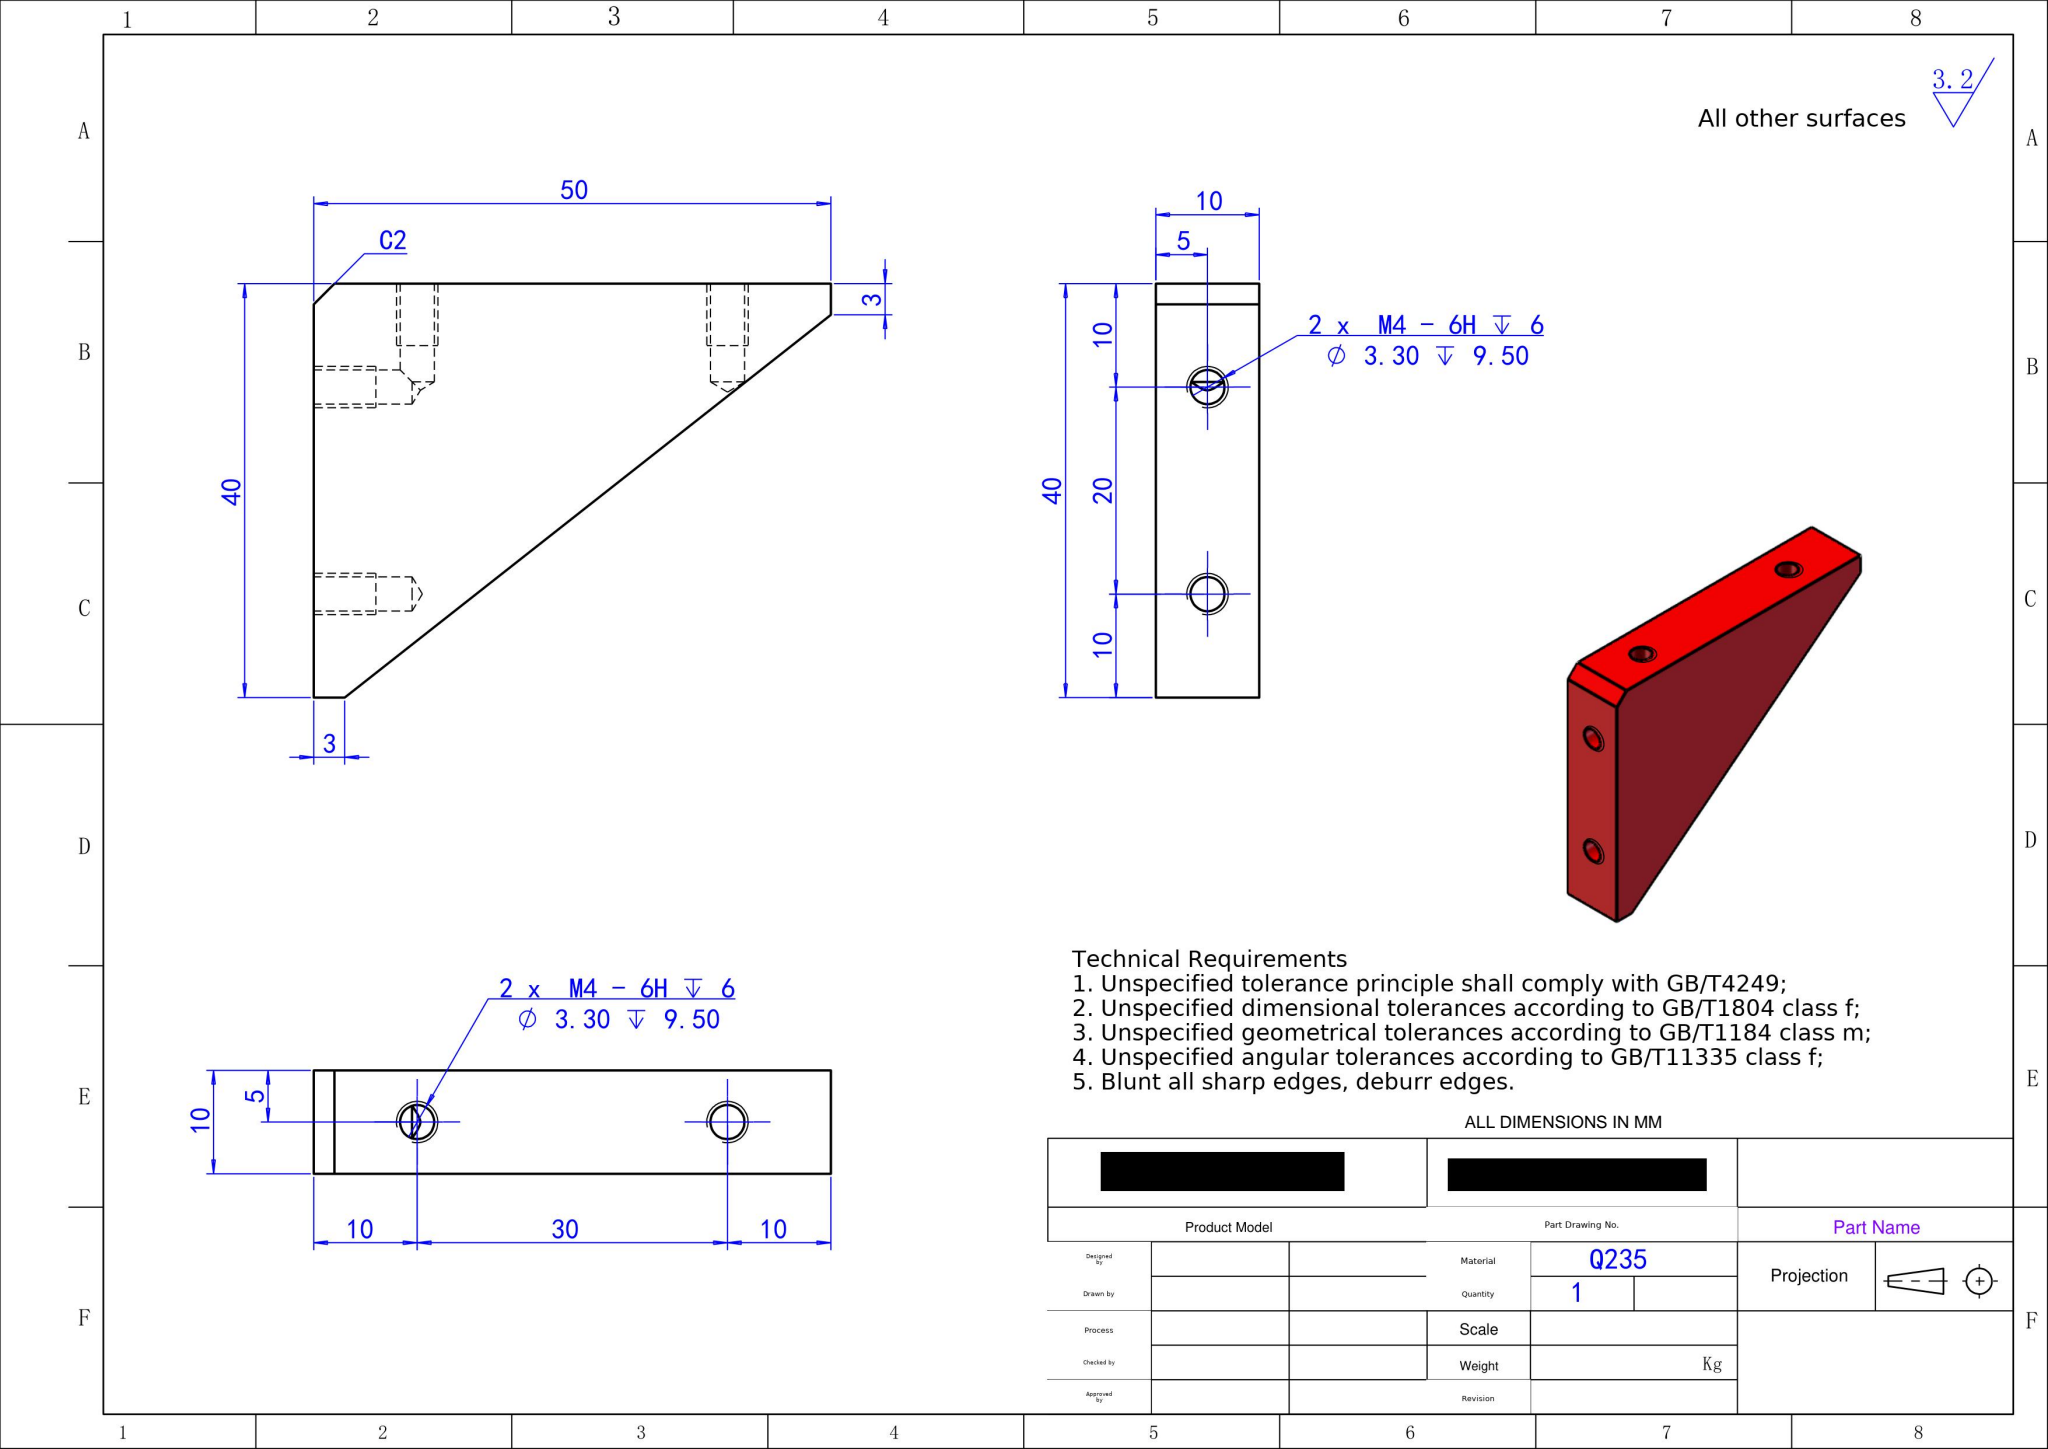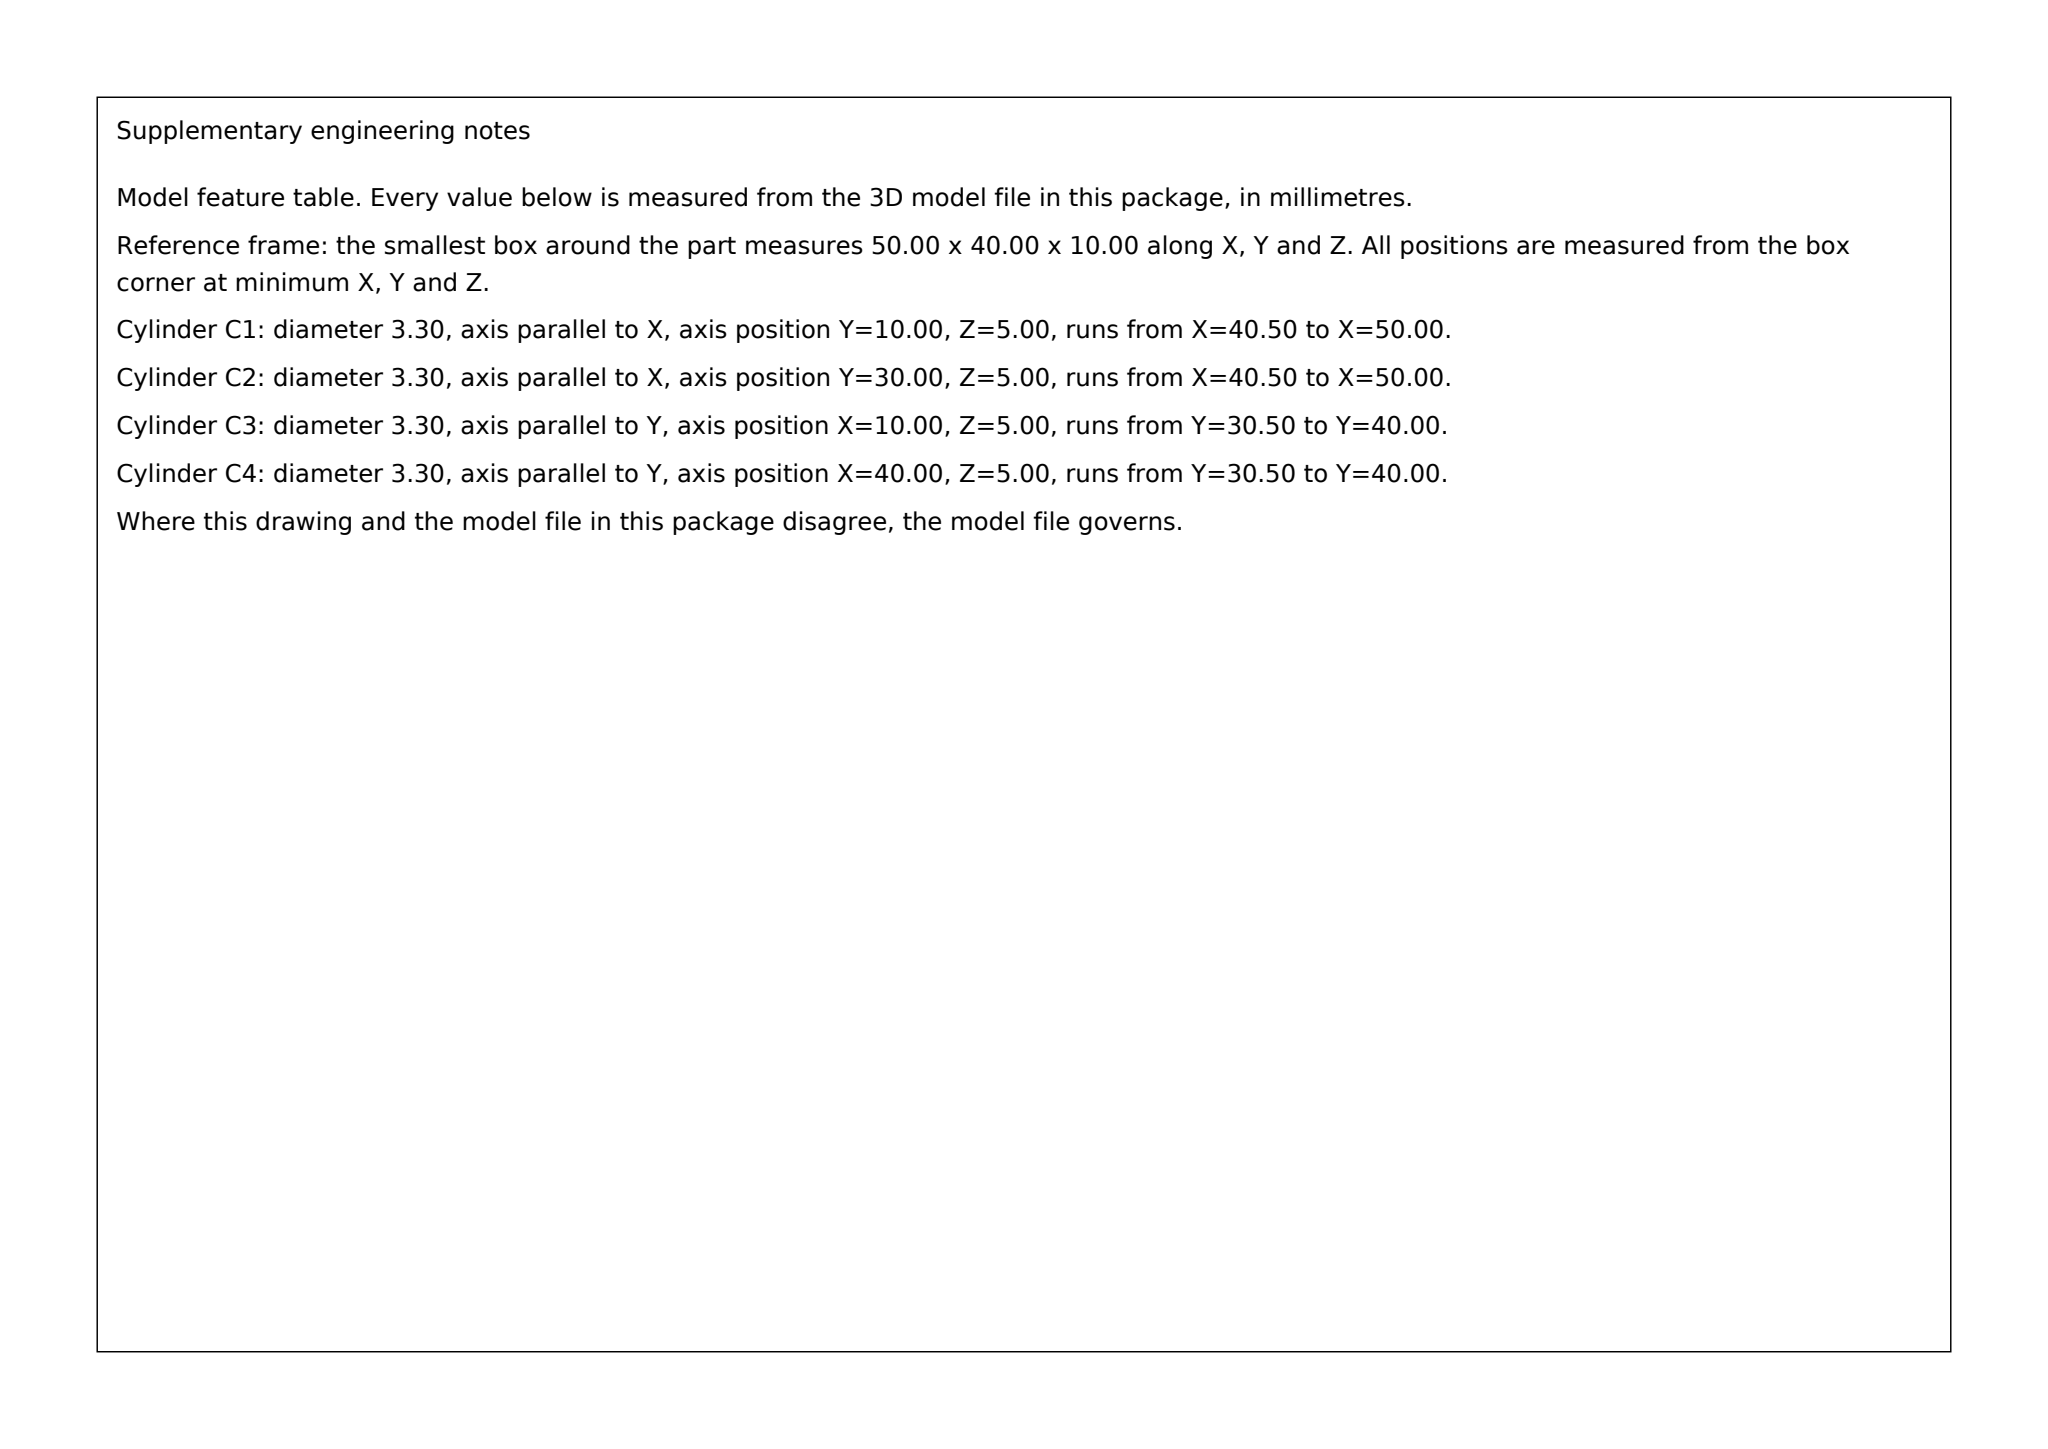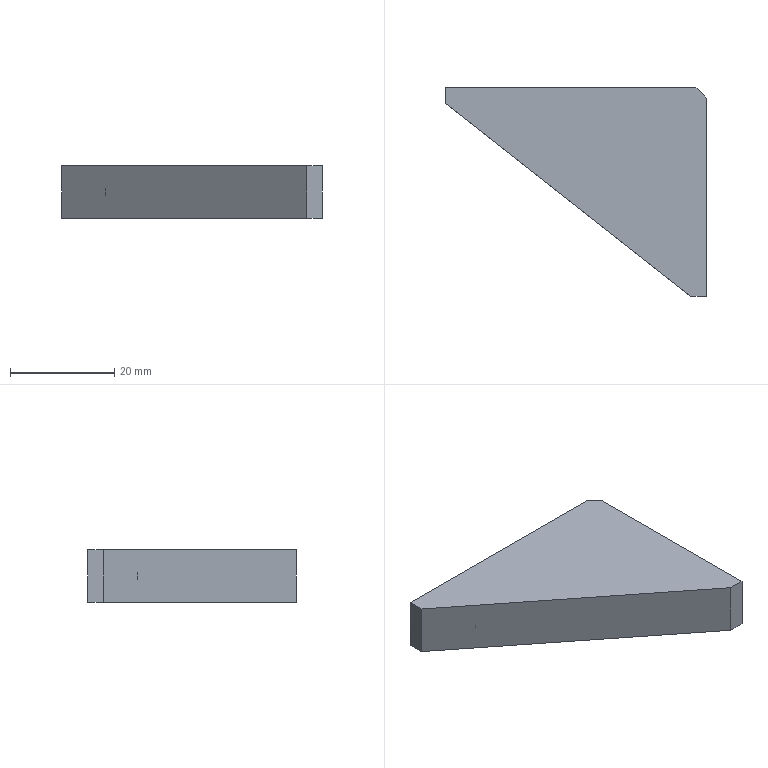Part | SolidWorks | mm | 1 solid | 26 faces | box 50 x 40 x 10 mm | volume 10953 mm3 | cone 10 | cylinder 8 | plane 8 | commonest cylinder face diameters 3.3 x8
build123d program:
from build123d import *

# Parameters (mm, degrees)
BOSS_EXTRUDE1_DEPTH   = 5
M4_TAPPED_HOLE1_D     = 3.3
M4_TAPPED_HOLE1_DEPTH = 9.5
M4_TAPPED_HOLE1_TIP   = 0.9914
M4_TAPPED_HOLE2_D     = 3.3
M4_TAPPED_HOLE2_DEPTH = 9.5
M4_TAPPED_HOLE2_TIP   = 0.9914
CHAMFER1_SIZE         = 2


with BuildPart() as part:
    # Sketch1 → Boss-Extrude1 (new, symmetric)
    with BuildSketch(Plane.XY):
        Polygon((-50, 0), (-50, -3), (-3, -40), (0, -40), (0, 0), align=None)
    extrude(amount=BOSS_EXTRUDE1_DEPTH, both=True)

    # M4 Tapped Hole1
    with Locations(Plane(origin=(0, 0, 0), x_dir=(1, 0, 0), z_dir=(0, 1, 0))):
        with Locations((-40, 0), (-10, 0)):
            Hole(M4_TAPPED_HOLE1_D / 2, depth=M4_TAPPED_HOLE1_DEPTH)
            with Locations((0, 0, -(M4_TAPPED_HOLE1_DEPTH + M4_TAPPED_HOLE1_TIP / 2))):  # 118° drill point
                Cone(0, M4_TAPPED_HOLE1_D / 2, M4_TAPPED_HOLE1_TIP, mode=Mode.SUBTRACT)

    # M4 Tapped Hole2
    with Locations(Plane(origin=(0, 0, 0), x_dir=(0, 0, -1), z_dir=(1, 0, 0))):
        with Locations((0, -10), (0, -30)):
            Hole(M4_TAPPED_HOLE2_D / 2, depth=M4_TAPPED_HOLE2_DEPTH)
            with Locations((0, 0, -(M4_TAPPED_HOLE2_DEPTH + M4_TAPPED_HOLE2_TIP / 2))):  # 118° drill point
                Cone(0, M4_TAPPED_HOLE2_D / 2, M4_TAPPED_HOLE2_TIP, mode=Mode.SUBTRACT)

    # Chamfer1
    chamfer1_edges = [part.edges().sort_by_distance(p)[0] for p in [
        (0, 0, 0),
    ]]
    chamfer(chamfer1_edges, length=CHAMFER1_SIZE)


solid = part.part
STEP:
#1=CARTESIAN_POINT('',(-10.,-10.,0.8179));
#2=VERTEX_POINT('',#1);
#3=CARTESIAN_POINT('',(-10.,-10.,-0.8179));
#4=VERTEX_POINT('',#3);
#5=CARTESIAN_POINT('',(-10.,-10.,0.8179));
#6=CARTESIAN_POINT('',(-10.072,-10.072,0.6979));
#7=CARTESIAN_POINT('',(-10.142,-10.142,0.5744));
#8=CARTESIAN_POINT('',(-10.23,-10.23,0.3745));
#9=CARTESIAN_POINT('',(-10.256,-10.256,0.3058));
#10=CARTESIAN_POINT('',(-10.294,-10.294,0.1596));
#11=CARTESIAN_POINT('',(-10.307,-10.307,0.08021));
#12=CARTESIAN_POINT('',(-10.307,-10.307,-0.07708));
#13=CARTESIAN_POINT('',(-10.295,-10.295,-0.1564));
#14=CARTESIAN_POINT('',(-10.256,-10.256,-0.3047));
#15=CARTESIAN_POINT('',(-10.229,-10.229,-0.3753));
#16=CARTESIAN_POINT('',(-10.141,-10.141,-0.5754));
#17=CARTESIAN_POINT('',(-10.072,-10.072,-0.698));
#18=CARTESIAN_POINT('',(-10.,-10.,-0.8179));
#19=B_SPLINE_CURVE_WITH_KNOTS('',3,(#5,#6,#7,#8,#9,#10,#11,#12,#13,#14,#15,#16,#17,#18),.UNSPECIFIED.,.F.,.F.,(4,2,2,2,2,2,4),(0.001035,0.001506,0.001742,0.001978,0.002213,0.002449,0.002921),.UNSPECIFIED.);
#20=EDGE_CURVE('',#2,#4,#19,.T.);
#21=ORIENTED_EDGE('',*,*,#20,.F.);
#22=CARTESIAN_POINT('',(-9.5,-10.,1.65));
#23=VERTEX_POINT('',#22);
#24=CARTESIAN_POINT('',(-9.5,-10.,1.65));
#25=DIRECTION('',(0.515,0.,0.8572));
#26=VECTOR('',#25,1000.);
#27=LINE('',#24,#26);
#28=EDGE_CURVE('',#2,#23,#27,.T.);
#29=ORIENTED_EDGE('',*,*,#28,.T.);
#30=CARTESIAN_POINT('',(-9.5,-10.,-1.65));
#31=VERTEX_POINT('',#30);
#32=CARTESIAN_POINT('',(-9.5,-10.,0.));
#33=DIRECTION('',(1.,0.,0.));
#34=DIRECTION('',(0.,0.,-1.));
#35=AXIS2_PLACEMENT_3D('',#32,#33,#34);
#36=CIRCLE('',#35,1.65);
#37=EDGE_CURVE('',#23,#31,#36,.T.);
#38=ORIENTED_EDGE('',*,*,#37,.T.);
#39=CARTESIAN_POINT('',(-9.5,-10.,-1.65));
#40=DIRECTION('',(0.515,0.,-0.8572));
#41=VECTOR('',#40,1000.);
#42=LINE('',#39,#41);
#43=EDGE_CURVE('',#4,#31,#42,.T.);
#44=ORIENTED_EDGE('',*,*,#43,.F.);
#45=EDGE_LOOP('',(#21,#29,#38,#44));
#46=FACE_OUTER_BOUND('',#45,.T.);
#47=CARTESIAN_POINT('',(-9.5,-10.,0.));
#48=DIRECTION('',(1.,0.,0.));
#49=DIRECTION('',(0.,0.,-1.));
#50=AXIS2_PLACEMENT_3D('',#47,#48,#49);
#51=CONICAL_SURFACE('',#50,1.65,1.03);
#52=ADVANCED_FACE('',(#46),#51,.F.);
#53=CARTESIAN_POINT('',(-9.5,-9.5,-1.572));
#54=VERTEX_POINT('',#53);
#55=CARTESIAN_POINT('',(-10.,-10.,-0.8179));
#56=CARTESIAN_POINT('',(-9.842,-9.842,-1.081));
#57=CARTESIAN_POINT('',(-9.672,-9.672,-1.327));
#58=CARTESIAN_POINT('',(-9.5,-9.5,-1.572));
#59=B_SPLINE_CURVE_WITH_KNOTS('',3,(#55,#56,#57,#58),.UNSPECIFIED.,.F.,.F.,(4,4),(0.002921,0.003954),.UNSPECIFIED.);
#60=EDGE_CURVE('',#4,#54,#59,.T.);
#61=ORIENTED_EDGE('',*,*,#60,.F.);
#62=ORIENTED_EDGE('',*,*,#43,.T.);
#63=CARTESIAN_POINT('',(-9.5,-10.,0.));
#64=DIRECTION('',(1.,0.,0.));
#65=DIRECTION('',(0.,0.,-1.));
#66=AXIS2_PLACEMENT_3D('',#63,#64,#65);
#67=CIRCLE('',#66,1.65);
#68=EDGE_CURVE('',#31,#54,#67,.T.);
#69=ORIENTED_EDGE('',*,*,#68,.T.);
#70=EDGE_LOOP('',(#61,#62,#69));
#71=FACE_OUTER_BOUND('',#70,.T.);
#72=CARTESIAN_POINT('',(-9.5,-10.,0.));
#73=DIRECTION('',(1.,0.,0.));
#74=DIRECTION('',(0.,0.,-1.));
#75=AXIS2_PLACEMENT_3D('',#72,#73,#74);
#76=CONICAL_SURFACE('',#75,1.65,1.03);
#77=ADVANCED_FACE('',(#71),#76,.F.);
#78=ORIENTED_EDGE('',*,*,#37,.F.);
#79=CARTESIAN_POINT('',(0.,-10.,1.65));
#80=VERTEX_POINT('',#79);
#81=CARTESIAN_POINT('',(0.,-10.,1.65));
#82=DIRECTION('',(1.,0.,0.));
#83=VECTOR('',#82,1000.);
#84=LINE('',#81,#83);
#85=EDGE_CURVE('',#23,#80,#84,.T.);
#86=ORIENTED_EDGE('',*,*,#85,.T.);
#87=CARTESIAN_POINT('',(0.,-10.,-1.65));
#88=VERTEX_POINT('',#87);
#89=CARTESIAN_POINT('',(0.,-10.,0.));
#90=DIRECTION('',(1.,0.,0.));
#91=DIRECTION('',(0.,0.,-1.));
#92=AXIS2_PLACEMENT_3D('',#89,#90,#91);
#93=CIRCLE('',#92,1.65);
#94=EDGE_CURVE('',#80,#88,#93,.T.);
#95=ORIENTED_EDGE('',*,*,#94,.T.);
#96=CARTESIAN_POINT('',(0.,-10.,-1.65));
#97=DIRECTION('',(1.,0.,0.));
#98=VECTOR('',#97,1000.);
#99=LINE('',#96,#98);
#100=EDGE_CURVE('',#31,#88,#99,.T.);
#101=ORIENTED_EDGE('',*,*,#100,.F.);
#102=EDGE_LOOP('',(#78,#86,#95,#101));
#103=FACE_OUTER_BOUND('',#102,.T.);
#104=CARTESIAN_POINT('',(0.,-10.,0.));
#105=DIRECTION('',(1.,0.,0.));
#106=DIRECTION('',(0.,0.,-1.));
#107=AXIS2_PLACEMENT_3D('',#104,#105,#106);
#108=CYLINDRICAL_SURFACE('',#107,1.65);
#109=ADVANCED_FACE('',(#103),#108,.F.);
#110=CARTESIAN_POINT('',(-9.5,-30.,1.65));
#111=VERTEX_POINT('',#110);
#112=CARTESIAN_POINT('',(-9.5,-30.,-1.65));
#113=VERTEX_POINT('',#112);
#114=CARTESIAN_POINT('',(-9.5,-30.,0.));
#115=DIRECTION('',(1.,0.,0.));
#116=DIRECTION('',(0.,0.,-1.));
#117=AXIS2_PLACEMENT_3D('',#114,#115,#116);
#118=CIRCLE('',#117,1.65);
#119=EDGE_CURVE('',#111,#113,#118,.T.);
#120=ORIENTED_EDGE('',*,*,#119,.F.);
#121=CARTESIAN_POINT('',(0.,-30.,1.65));
#122=VERTEX_POINT('',#121);
#123=CARTESIAN_POINT('',(0.,-30.,1.65));
#124=DIRECTION('',(1.,0.,0.));
#125=VECTOR('',#124,1000.);
#126=LINE('',#123,#125);
#127=EDGE_CURVE('',#111,#122,#126,.T.);
#128=ORIENTED_EDGE('',*,*,#127,.T.);
#129=CARTESIAN_POINT('',(0.,-30.,-1.65));
#130=VERTEX_POINT('',#129);
#131=CARTESIAN_POINT('',(0.,-30.,0.));
#132=DIRECTION('',(1.,0.,0.));
#133=DIRECTION('',(0.,0.,-1.));
#134=AXIS2_PLACEMENT_3D('',#131,#132,#133);
#135=CIRCLE('',#134,1.65);
#136=EDGE_CURVE('',#122,#130,#135,.T.);
#137=ORIENTED_EDGE('',*,*,#136,.T.);
#138=CARTESIAN_POINT('',(0.,-30.,-1.65));
#139=DIRECTION('',(1.,0.,0.));
#140=VECTOR('',#139,1000.);
#141=LINE('',#138,#140);
#142=EDGE_CURVE('',#113,#130,#141,.T.);
#143=ORIENTED_EDGE('',*,*,#142,.F.);
#144=EDGE_LOOP('',(#120,#128,#137,#143));
#145=FACE_OUTER_BOUND('',#144,.T.);
#146=CARTESIAN_POINT('',(0.,-30.,0.));
#147=DIRECTION('',(1.,0.,0.));
#148=DIRECTION('',(0.,0.,-1.));
#149=AXIS2_PLACEMENT_3D('',#146,#147,#148);
#150=CYLINDRICAL_SURFACE('',#149,1.65);
#151=ADVANCED_FACE('',(#145),#150,.F.);
#152=CARTESIAN_POINT('',(-10.491,-30.,0.));
#153=VERTEX_POINT('',#152);
#154=CARTESIAN_POINT('',(-9.5,-30.,-1.65));
#155=DIRECTION('',(0.515,0.,-0.8572));
#156=VECTOR('',#155,1000.);
#157=LINE('',#154,#156);
#158=EDGE_CURVE('',#153,#113,#157,.T.);
#159=ORIENTED_EDGE('',*,*,#158,.F.);
#160=CARTESIAN_POINT('',(-9.5,-30.,1.65));
#161=DIRECTION('',(0.515,0.,0.8572));
#162=VECTOR('',#161,1000.);
#163=LINE('',#160,#162);
#164=EDGE_CURVE('',#153,#111,#163,.T.);
#165=ORIENTED_EDGE('',*,*,#164,.T.);
#166=ORIENTED_EDGE('',*,*,#119,.T.);
#167=EDGE_LOOP('',(#159,#165,#166));
#168=FACE_OUTER_BOUND('',#167,.T.);
#169=CARTESIAN_POINT('',(-9.5,-30.,0.));
#170=DIRECTION('',(1.,0.,0.));
#171=DIRECTION('',(0.,0.,-1.));
#172=AXIS2_PLACEMENT_3D('',#169,#170,#171);
#173=CONICAL_SURFACE('',#172,1.65,1.03);
#174=ADVANCED_FACE('',(#168),#173,.F.);
#175=CARTESIAN_POINT('',(-40.,-9.5,-1.65));
#176=VERTEX_POINT('',#175);
#177=CARTESIAN_POINT('',(-40.,-9.5,1.65));
#178=VERTEX_POINT('',#177);
#179=CARTESIAN_POINT('',(-40.,-9.5,0.));
#180=DIRECTION('',(0.,1.,0.));
#181=DIRECTION('',(0.,0.,1.));
#182=AXIS2_PLACEMENT_3D('',#179,#180,#181);
#183=CIRCLE('',#182,1.65);
#184=EDGE_CURVE('',#176,#178,#183,.T.);
#185=ORIENTED_EDGE('',*,*,#184,.F.);
#186=CARTESIAN_POINT('',(-40.,-0.,-1.65));
#187=VERTEX_POINT('',#186);
#188=CARTESIAN_POINT('',(-40.,-0.,-1.65));
#189=DIRECTION('',(0.,1.,0.));
#190=VECTOR('',#189,1000.);
#191=LINE('',#188,#190);
#192=EDGE_CURVE('',#176,#187,#191,.T.);
#193=ORIENTED_EDGE('',*,*,#192,.T.);
#194=CARTESIAN_POINT('',(-40.,-0.,1.65));
#195=VERTEX_POINT('',#194);
#196=CARTESIAN_POINT('',(-40.,-0.,0.));
#197=DIRECTION('',(0.,1.,0.));
#198=DIRECTION('',(0.,0.,1.));
#199=AXIS2_PLACEMENT_3D('',#196,#197,#198);
#200=CIRCLE('',#199,1.65);
#201=EDGE_CURVE('',#187,#195,#200,.T.);
#202=ORIENTED_EDGE('',*,*,#201,.T.);
#203=CARTESIAN_POINT('',(-40.,-0.,1.65));
#204=DIRECTION('',(0.,1.,0.));
#205=VECTOR('',#204,1000.);
#206=LINE('',#203,#205);
#207=EDGE_CURVE('',#178,#195,#206,.T.);
#208=ORIENTED_EDGE('',*,*,#207,.F.);
#209=EDGE_LOOP('',(#185,#193,#202,#208));
#210=FACE_OUTER_BOUND('',#209,.T.);
#211=CARTESIAN_POINT('',(-40.,-0.,0.));
#212=DIRECTION('',(0.,1.,0.));
#213=DIRECTION('',(0.,0.,1.));
#214=AXIS2_PLACEMENT_3D('',#211,#212,#213);
#215=CYLINDRICAL_SURFACE('',#214,1.65);
#216=ADVANCED_FACE('',(#210),#215,.F.);
#217=CARTESIAN_POINT('',(-40.,-10.491,0.));
#218=VERTEX_POINT('',#217);
#219=CARTESIAN_POINT('',(-40.,-9.5,1.65));
#220=DIRECTION('',(0.,0.515,0.8572));
#221=VECTOR('',#220,1000.);
#222=LINE('',#219,#221);
#223=EDGE_CURVE('',#218,#178,#222,.T.);
#224=ORIENTED_EDGE('',*,*,#223,.F.);
#225=CARTESIAN_POINT('',(-40.,-9.5,-1.65));
#226=DIRECTION('',(0.,0.515,-0.8572));
#227=VECTOR('',#226,1000.);
#228=LINE('',#225,#227);
#229=EDGE_CURVE('',#218,#176,#228,.T.);
#230=ORIENTED_EDGE('',*,*,#229,.T.);
#231=ORIENTED_EDGE('',*,*,#184,.T.);
#232=EDGE_LOOP('',(#224,#230,#231));
#233=FACE_OUTER_BOUND('',#232,.T.);
#234=CARTESIAN_POINT('',(-40.,-9.5,0.));
#235=DIRECTION('',(0.,1.,0.));
#236=DIRECTION('',(0.,0.,1.));
#237=AXIS2_PLACEMENT_3D('',#234,#235,#236);
#238=CONICAL_SURFACE('',#237,1.65,1.03);
#239=ADVANCED_FACE('',(#233),#238,.F.);
#240=CARTESIAN_POINT('',(-10.,-9.5,-1.65));
#241=VERTEX_POINT('',#240);
#242=CARTESIAN_POINT('',(-10.,-9.5,1.65));
#243=VERTEX_POINT('',#242);
#244=CARTESIAN_POINT('',(-10.,-9.5,0.));
#245=DIRECTION('',(0.,1.,0.));
#246=DIRECTION('',(0.,0.,1.));
#247=AXIS2_PLACEMENT_3D('',#244,#245,#246);
#248=CIRCLE('',#247,1.65);
#249=EDGE_CURVE('',#241,#243,#248,.T.);
#250=ORIENTED_EDGE('',*,*,#249,.F.);
#251=CARTESIAN_POINT('',(-10.,0.,-1.65));
#252=VERTEX_POINT('',#251);
#253=CARTESIAN_POINT('',(-10.,0.,-1.65));
#254=DIRECTION('',(0.,1.,0.));
#255=VECTOR('',#254,1000.);
#256=LINE('',#253,#255);
#257=EDGE_CURVE('',#241,#252,#256,.T.);
#258=ORIENTED_EDGE('',*,*,#257,.T.);
#259=CARTESIAN_POINT('',(-10.,0.,1.65));
#260=VERTEX_POINT('',#259);
#261=CARTESIAN_POINT('',(-10.,0.,0.));
#262=DIRECTION('',(0.,1.,0.));
#263=DIRECTION('',(0.,0.,1.));
#264=AXIS2_PLACEMENT_3D('',#261,#262,#263);
#265=CIRCLE('',#264,1.65);
#266=EDGE_CURVE('',#252,#260,#265,.T.);
#267=ORIENTED_EDGE('',*,*,#266,.T.);
#268=CARTESIAN_POINT('',(-10.,0.,1.65));
#269=DIRECTION('',(0.,1.,0.));
#270=VECTOR('',#269,1000.);
#271=LINE('',#268,#270);
#272=EDGE_CURVE('',#243,#260,#271,.T.);
#273=ORIENTED_EDGE('',*,*,#272,.F.);
#274=EDGE_LOOP('',(#250,#258,#267,#273));
#275=FACE_OUTER_BOUND('',#274,.T.);
#276=CARTESIAN_POINT('',(-10.,0.,0.));
#277=DIRECTION('',(0.,1.,0.));
#278=DIRECTION('',(0.,0.,1.));
#279=AXIS2_PLACEMENT_3D('',#276,#277,#278);
#280=CYLINDRICAL_SURFACE('',#279,1.65);
#281=ADVANCED_FACE('',(#275),#280,.F.);
#282=ORIENTED_EDGE('',*,*,#20,.T.);
#283=CARTESIAN_POINT('',(-10.,-9.5,-1.65));
#284=DIRECTION('',(0.,0.515,-0.8572));
#285=VECTOR('',#284,1000.);
#286=LINE('',#283,#285);
#287=EDGE_CURVE('',#4,#241,#286,.T.);
#288=ORIENTED_EDGE('',*,*,#287,.T.);
#289=ORIENTED_EDGE('',*,*,#249,.T.);
#290=CARTESIAN_POINT('',(-10.,-9.5,1.65));
#291=DIRECTION('',(0.,0.515,0.8572));
#292=VECTOR('',#291,1000.);
#293=LINE('',#290,#292);
#294=EDGE_CURVE('',#2,#243,#293,.T.);
#295=ORIENTED_EDGE('',*,*,#294,.F.);
#296=EDGE_LOOP('',(#282,#288,#289,#295));
#297=FACE_OUTER_BOUND('',#296,.T.);
#298=CARTESIAN_POINT('',(-10.,-9.5,0.));
#299=DIRECTION('',(0.,1.,0.));
#300=DIRECTION('',(0.,0.,1.));
#301=AXIS2_PLACEMENT_3D('',#298,#299,#300);
#302=CONICAL_SURFACE('',#301,1.65,1.03);
#303=ADVANCED_FACE('',(#297),#302,.F.);
#304=CARTESIAN_POINT('',(-9.5,-9.5,1.572));
#305=VERTEX_POINT('',#304);
#306=CARTESIAN_POINT('',(-9.5,-9.5,1.572));
#307=CARTESIAN_POINT('',(-9.672,-9.672,1.327));
#308=CARTESIAN_POINT('',(-9.842,-9.842,1.081));
#309=CARTESIAN_POINT('',(-10.,-10.,0.8179));
#310=B_SPLINE_CURVE_WITH_KNOTS('',3,(#306,#307,#308,#309),.UNSPECIFIED.,.F.,.F.,(4,4),(0.0000004,0.001035),.UNSPECIFIED.);
#311=EDGE_CURVE('',#305,#2,#310,.T.);
#312=ORIENTED_EDGE('',*,*,#311,.T.);
#313=ORIENTED_EDGE('',*,*,#294,.T.);
#314=CARTESIAN_POINT('',(-10.,-9.5,0.));
#315=DIRECTION('',(0.,1.,0.));
#316=DIRECTION('',(0.,0.,1.));
#317=AXIS2_PLACEMENT_3D('',#314,#315,#316);
#318=CIRCLE('',#317,1.65);
#319=EDGE_CURVE('',#243,#305,#318,.T.);
#320=ORIENTED_EDGE('',*,*,#319,.T.);
#321=EDGE_LOOP('',(#312,#313,#320));
#322=FACE_OUTER_BOUND('',#321,.T.);
#323=CARTESIAN_POINT('',(-10.,-9.5,0.));
#324=DIRECTION('',(0.,1.,0.));
#325=DIRECTION('',(0.,0.,1.));
#326=AXIS2_PLACEMENT_3D('',#323,#324,#325);
#327=CONICAL_SURFACE('',#326,1.65,1.03);
#328=ADVANCED_FACE('',(#322),#327,.F.);
#329=CARTESIAN_POINT('',(-40.,-0.,0.));
#330=DIRECTION('',(0.,1.,0.));
#331=DIRECTION('',(0.,0.,1.));
#332=AXIS2_PLACEMENT_3D('',#329,#330,#331);
#333=CIRCLE('',#332,1.65);
#334=EDGE_CURVE('',#195,#187,#333,.T.);
#335=ORIENTED_EDGE('',*,*,#334,.F.);
#336=ORIENTED_EDGE('',*,*,#201,.F.);
#337=EDGE_LOOP('',(#335,#336));
#338=FACE_BOUND('',#337,.T.);
#339=CARTESIAN_POINT('',(-10.,0.,0.));
#340=DIRECTION('',(0.,1.,0.));
#341=DIRECTION('',(0.,0.,1.));
#342=AXIS2_PLACEMENT_3D('',#339,#340,#341);
#343=CIRCLE('',#342,1.65);
#344=EDGE_CURVE('',#260,#252,#343,.T.);
#345=ORIENTED_EDGE('',*,*,#344,.F.);
#346=ORIENTED_EDGE('',*,*,#266,.F.);
#347=EDGE_LOOP('',(#345,#346));
#348=FACE_BOUND('',#347,.T.);
#349=CARTESIAN_POINT('',(-2.,0.,5.));
#350=VERTEX_POINT('',#349);
#351=CARTESIAN_POINT('',(-50.,-0.,5.));
#352=VERTEX_POINT('',#351);
#353=CARTESIAN_POINT('',(0.,0.,5.));
#354=DIRECTION('',(-1.,-0.,0.));
#355=VECTOR('',#354,1000.);
#356=LINE('',#353,#355);
#357=EDGE_CURVE('',#350,#352,#356,.T.);
#358=ORIENTED_EDGE('',*,*,#357,.F.);
#359=CARTESIAN_POINT('',(-2.,0.,-5.));
#360=VERTEX_POINT('',#359);
#361=CARTESIAN_POINT('',(-2.,0.,-5.));
#362=DIRECTION('',(0.,0.,-1.));
#363=VECTOR('',#362,1000.);
#364=LINE('',#361,#363);
#365=EDGE_CURVE('',#350,#360,#364,.T.);
#366=ORIENTED_EDGE('',*,*,#365,.T.);
#367=CARTESIAN_POINT('',(-50.,-0.,-5.));
#368=VERTEX_POINT('',#367);
#369=CARTESIAN_POINT('',(0.,0.,-5.));
#370=DIRECTION('',(-1.,-0.,0.));
#371=VECTOR('',#370,1000.);
#372=LINE('',#369,#371);
#373=EDGE_CURVE('',#360,#368,#372,.T.);
#374=ORIENTED_EDGE('',*,*,#373,.T.);
#375=CARTESIAN_POINT('',(-50.,-0.,5.));
#376=DIRECTION('',(0.,0.,-1.));
#377=VECTOR('',#376,1000.);
#378=LINE('',#375,#377);
#379=EDGE_CURVE('',#352,#368,#378,.T.);
#380=ORIENTED_EDGE('',*,*,#379,.F.);
#381=EDGE_LOOP('',(#358,#366,#374,#380));
#382=FACE_OUTER_BOUND('',#381,.T.);
#383=CARTESIAN_POINT('',(0.,0.,5.));
#384=DIRECTION('',(0.,-1.,0.));
#385=DIRECTION('',(1.,0.,0.));
#386=AXIS2_PLACEMENT_3D('',#383,#384,#385);
#387=PLANE('',#386);
#388=ADVANCED_FACE('',(#338,#348,#382),#387,.F.);
#389=CARTESIAN_POINT('',(-50.,-3.,-5.));
#390=VERTEX_POINT('',#389);
#391=CARTESIAN_POINT('',(-50.,-0.,-5.));
#392=DIRECTION('',(0.,-1.,0.));
#393=VECTOR('',#392,1000.);
#394=LINE('',#391,#393);
#395=EDGE_CURVE('',#368,#390,#394,.T.);
#396=ORIENTED_EDGE('',*,*,#395,.T.);
#397=CARTESIAN_POINT('',(-50.,-3.,5.));
#398=VERTEX_POINT('',#397);
#399=CARTESIAN_POINT('',(-50.,-3.,5.));
#400=DIRECTION('',(0.,0.,-1.));
#401=VECTOR('',#400,1000.);
#402=LINE('',#399,#401);
#403=EDGE_CURVE('',#398,#390,#402,.T.);
#404=ORIENTED_EDGE('',*,*,#403,.F.);
#405=CARTESIAN_POINT('',(-50.,-0.,5.));
#406=DIRECTION('',(0.,-1.,0.));
#407=VECTOR('',#406,1000.);
#408=LINE('',#405,#407);
#409=EDGE_CURVE('',#352,#398,#408,.T.);
#410=ORIENTED_EDGE('',*,*,#409,.F.);
#411=ORIENTED_EDGE('',*,*,#379,.T.);
#412=EDGE_LOOP('',(#396,#404,#410,#411));
#413=FACE_OUTER_BOUND('',#412,.T.);
#414=CARTESIAN_POINT('',(-50.,-0.,5.));
#415=DIRECTION('',(1.,0.,0.));
#416=DIRECTION('',(-0.,1.,0.));
#417=AXIS2_PLACEMENT_3D('',#414,#415,#416);
#418=PLANE('',#417);
#419=ADVANCED_FACE('',(#413),#418,.F.);
#420=CARTESIAN_POINT('',(-3.,-40.,-5.));
#421=VERTEX_POINT('',#420);
#422=CARTESIAN_POINT('',(-20.589,-26.153,-5.));
#423=DIRECTION('',(0.7857,-0.6186,0.));
#424=VECTOR('',#423,1000.);
#425=LINE('',#422,#424);
#426=EDGE_CURVE('',#390,#421,#425,.T.);
#427=ORIENTED_EDGE('',*,*,#426,.T.);
#428=CARTESIAN_POINT('',(-3.,-40.,5.));
#429=VERTEX_POINT('',#428);
#430=CARTESIAN_POINT('',(-3.,-40.,5.));
#431=DIRECTION('',(0.,0.,-1.));
#432=VECTOR('',#431,1000.);
#433=LINE('',#430,#432);
#434=EDGE_CURVE('',#429,#421,#433,.T.);
#435=ORIENTED_EDGE('',*,*,#434,.F.);
#436=CARTESIAN_POINT('',(-20.589,-26.153,5.));
#437=DIRECTION('',(0.7857,-0.6186,0.));
#438=VECTOR('',#437,1000.);
#439=LINE('',#436,#438);
#440=EDGE_CURVE('',#398,#429,#439,.T.);
#441=ORIENTED_EDGE('',*,*,#440,.F.);
#442=ORIENTED_EDGE('',*,*,#403,.T.);
#443=EDGE_LOOP('',(#427,#435,#441,#442));
#444=FACE_OUTER_BOUND('',#443,.T.);
#445=CARTESIAN_POINT('',(-20.589,-26.153,5.));
#446=DIRECTION('',(0.6186,0.7857,0.));
#447=DIRECTION('',(-0.7857,0.6186,0.));
#448=AXIS2_PLACEMENT_3D('',#445,#446,#447);
#449=PLANE('',#448);
#450=ADVANCED_FACE('',(#444),#449,.F.);
#451=CARTESIAN_POINT('',(0.,-40.,-5.));
#452=VERTEX_POINT('',#451);
#453=CARTESIAN_POINT('',(0.,-40.,-5.));
#454=DIRECTION('',(-1.,-0.,0.));
#455=VECTOR('',#454,1000.);
#456=LINE('',#453,#455);
#457=EDGE_CURVE('',#452,#421,#456,.T.);
#458=ORIENTED_EDGE('',*,*,#457,.F.);
#459=CARTESIAN_POINT('',(0.,-40.,5.));
#460=VERTEX_POINT('',#459);
#461=CARTESIAN_POINT('',(0.,-40.,5.));
#462=DIRECTION('',(0.,0.,-1.));
#463=VECTOR('',#462,1000.);
#464=LINE('',#461,#463);
#465=EDGE_CURVE('',#460,#452,#464,.T.);
#466=ORIENTED_EDGE('',*,*,#465,.F.);
#467=CARTESIAN_POINT('',(0.,-40.,5.));
#468=DIRECTION('',(-1.,-0.,0.));
#469=VECTOR('',#468,1000.);
#470=LINE('',#467,#469);
#471=EDGE_CURVE('',#460,#429,#470,.T.);
#472=ORIENTED_EDGE('',*,*,#471,.T.);
#473=ORIENTED_EDGE('',*,*,#434,.T.);
#474=EDGE_LOOP('',(#458,#466,#472,#473));
#475=FACE_OUTER_BOUND('',#474,.T.);
#476=CARTESIAN_POINT('',(0.,-40.,5.));
#477=DIRECTION('',(0.,-1.,0.));
#478=DIRECTION('',(1.,0.,0.));
#479=AXIS2_PLACEMENT_3D('',#476,#477,#478);
#480=PLANE('',#479);
#481=ADVANCED_FACE('',(#475),#480,.T.);
#482=CARTESIAN_POINT('',(0.,-10.,0.));
#483=DIRECTION('',(1.,0.,0.));
#484=DIRECTION('',(0.,0.,-1.));
#485=AXIS2_PLACEMENT_3D('',#482,#483,#484);
#486=CIRCLE('',#485,1.65);
#487=EDGE_CURVE('',#88,#80,#486,.T.);
#488=ORIENTED_EDGE('',*,*,#487,.F.);
#489=ORIENTED_EDGE('',*,*,#94,.F.);
#490=EDGE_LOOP('',(#488,#489));
#491=FACE_BOUND('',#490,.T.);
#492=CARTESIAN_POINT('',(0.,-30.,0.));
#493=DIRECTION('',(1.,0.,0.));
#494=DIRECTION('',(0.,0.,-1.));
#495=AXIS2_PLACEMENT_3D('',#492,#493,#494);
#496=CIRCLE('',#495,1.65);
#497=EDGE_CURVE('',#130,#122,#496,.T.);
#498=ORIENTED_EDGE('',*,*,#497,.F.);
#499=ORIENTED_EDGE('',*,*,#136,.F.);
#500=EDGE_LOOP('',(#498,#499));
#501=FACE_BOUND('',#500,.T.);
#502=CARTESIAN_POINT('',(0.,-2.,-5.));
#503=VERTEX_POINT('',#502);
#504=CARTESIAN_POINT('',(0.,0.,-5.));
#505=DIRECTION('',(0.,-1.,0.));
#506=VECTOR('',#505,1000.);
#507=LINE('',#504,#506);
#508=EDGE_CURVE('',#503,#452,#507,.T.);
#509=ORIENTED_EDGE('',*,*,#508,.F.);
#510=CARTESIAN_POINT('',(0.,-2.,5.));
#511=VERTEX_POINT('',#510);
#512=CARTESIAN_POINT('',(0.,-2.,5.));
#513=DIRECTION('',(0.,0.,1.));
#514=VECTOR('',#513,1000.);
#515=LINE('',#512,#514);
#516=EDGE_CURVE('',#503,#511,#515,.T.);
#517=ORIENTED_EDGE('',*,*,#516,.T.);
#518=CARTESIAN_POINT('',(0.,0.,5.));
#519=DIRECTION('',(0.,-1.,0.));
#520=VECTOR('',#519,1000.);
#521=LINE('',#518,#520);
#522=EDGE_CURVE('',#511,#460,#521,.T.);
#523=ORIENTED_EDGE('',*,*,#522,.T.);
#524=ORIENTED_EDGE('',*,*,#465,.T.);
#525=EDGE_LOOP('',(#509,#517,#523,#524));
#526=FACE_OUTER_BOUND('',#525,.T.);
#527=CARTESIAN_POINT('',(0.,0.,5.));
#528=DIRECTION('',(1.,0.,0.));
#529=DIRECTION('',(-0.,1.,0.));
#530=AXIS2_PLACEMENT_3D('',#527,#528,#529);
#531=PLANE('',#530);
#532=ADVANCED_FACE('',(#491,#501,#526),#531,.T.);
#533=ORIENTED_EDGE('',*,*,#522,.F.);
#534=CARTESIAN_POINT('',(-1.,-1.,5.));
#535=DIRECTION('',(-0.7071,0.7071,0.));
#536=VECTOR('',#535,1000.);
#537=LINE('',#534,#536);
#538=EDGE_CURVE('',#511,#350,#537,.T.);
#539=ORIENTED_EDGE('',*,*,#538,.T.);
#540=ORIENTED_EDGE('',*,*,#357,.T.);
#541=ORIENTED_EDGE('',*,*,#409,.T.);
#542=ORIENTED_EDGE('',*,*,#440,.T.);
#543=ORIENTED_EDGE('',*,*,#471,.F.);
#544=EDGE_LOOP('',(#533,#539,#540,#541,#542,#543));
#545=FACE_OUTER_BOUND('',#544,.T.);
#546=CARTESIAN_POINT('',(0.,0.,5.));
#547=DIRECTION('',(0.,0.,1.));
#548=DIRECTION('',(1.,0.,0.));
#549=AXIS2_PLACEMENT_3D('',#546,#547,#548);
#550=PLANE('',#549);
#551=ADVANCED_FACE('',(#545),#550,.T.);
#552=ORIENTED_EDGE('',*,*,#373,.F.);
#553=CARTESIAN_POINT('',(-2.,0.,-5.));
#554=DIRECTION('',(0.7071,-0.7071,0.));
#555=VECTOR('',#554,1000.);
#556=LINE('',#553,#555);
#557=EDGE_CURVE('',#360,#503,#556,.T.);
#558=ORIENTED_EDGE('',*,*,#557,.T.);
#559=ORIENTED_EDGE('',*,*,#508,.T.);
#560=ORIENTED_EDGE('',*,*,#457,.T.);
#561=ORIENTED_EDGE('',*,*,#426,.F.);
#562=ORIENTED_EDGE('',*,*,#395,.F.);
#563=EDGE_LOOP('',(#552,#558,#559,#560,#561,#562));
#564=FACE_OUTER_BOUND('',#563,.T.);
#565=CARTESIAN_POINT('',(0.,0.,-5.));
#566=DIRECTION('',(0.,0.,1.));
#567=DIRECTION('',(1.,0.,0.));
#568=AXIS2_PLACEMENT_3D('',#565,#566,#567);
#569=PLANE('',#568);
#570=ADVANCED_FACE('',(#564),#569,.F.);
#571=ORIENTED_EDGE('',*,*,#287,.F.);
#572=ORIENTED_EDGE('',*,*,#60,.T.);
#573=CARTESIAN_POINT('',(-10.,-9.5,0.));
#574=DIRECTION('',(0.,1.,0.));
#575=DIRECTION('',(0.,0.,1.));
#576=AXIS2_PLACEMENT_3D('',#573,#574,#575);
#577=CIRCLE('',#576,1.65);
#578=EDGE_CURVE('',#54,#241,#577,.T.);
#579=ORIENTED_EDGE('',*,*,#578,.T.);
#580=EDGE_LOOP('',(#571,#572,#579));
#581=FACE_OUTER_BOUND('',#580,.T.);
#582=CARTESIAN_POINT('',(-10.,-9.5,0.));
#583=DIRECTION('',(0.,1.,0.));
#584=DIRECTION('',(0.,0.,1.));
#585=AXIS2_PLACEMENT_3D('',#582,#583,#584);
#586=CONICAL_SURFACE('',#585,1.65,1.03);
#587=ADVANCED_FACE('',(#581),#586,.F.);
#588=ORIENTED_EDGE('',*,*,#257,.F.);
#589=ORIENTED_EDGE('',*,*,#578,.F.);
#590=CARTESIAN_POINT('',(-9.5,-9.5,-1.572));
#591=CARTESIAN_POINT('',(-7.634,-7.634,-0.9791));
#592=CARTESIAN_POINT('',(-7.634,-7.634,0.9791));
#593=CARTESIAN_POINT('',(-9.5,-9.5,1.572));
#594=(BOUNDED_CURVE()B_SPLINE_CURVE(3,(#590,#591,#592,#593),.UNSPECIFIED.,.F.,.F.)B_SPLINE_CURVE_WITH_KNOTS((4,4),(5.02,7.546),.UNSPECIFIED.)CURVE()GEOMETRIC_REPRESENTATION_ITEM()RATIONAL_B_SPLINE_CURVE((1.,0.5354,0.5354,1.))REPRESENTATION_ITEM(''));
#595=EDGE_CURVE('',#54,#305,#594,.T.);
#596=ORIENTED_EDGE('',*,*,#595,.T.);
#597=ORIENTED_EDGE('',*,*,#319,.F.);
#598=ORIENTED_EDGE('',*,*,#272,.T.);
#599=ORIENTED_EDGE('',*,*,#344,.T.);
#600=EDGE_LOOP('',(#588,#589,#596,#597,#598,#599));
#601=FACE_OUTER_BOUND('',#600,.T.);
#602=CARTESIAN_POINT('',(-10.,0.,0.));
#603=DIRECTION('',(0.,1.,0.));
#604=DIRECTION('',(0.,0.,1.));
#605=AXIS2_PLACEMENT_3D('',#602,#603,#604);
#606=CYLINDRICAL_SURFACE('',#605,1.65);
#607=ADVANCED_FACE('',(#601),#606,.F.);
#608=ORIENTED_EDGE('',*,*,#229,.F.);
#609=ORIENTED_EDGE('',*,*,#223,.T.);
#610=CARTESIAN_POINT('',(-40.,-9.5,0.));
#611=DIRECTION('',(0.,1.,0.));
#612=DIRECTION('',(0.,0.,1.));
#613=AXIS2_PLACEMENT_3D('',#610,#611,#612);
#614=CIRCLE('',#613,1.65);
#615=EDGE_CURVE('',#178,#176,#614,.T.);
#616=ORIENTED_EDGE('',*,*,#615,.T.);
#617=EDGE_LOOP('',(#608,#609,#616));
#618=FACE_OUTER_BOUND('',#617,.T.);
#619=CARTESIAN_POINT('',(-40.,-9.5,0.));
#620=DIRECTION('',(0.,1.,0.));
#621=DIRECTION('',(0.,0.,1.));
#622=AXIS2_PLACEMENT_3D('',#619,#620,#621);
#623=CONICAL_SURFACE('',#622,1.65,1.03);
#624=ADVANCED_FACE('',(#618),#623,.F.);
#625=ORIENTED_EDGE('',*,*,#192,.F.);
#626=ORIENTED_EDGE('',*,*,#615,.F.);
#627=ORIENTED_EDGE('',*,*,#207,.T.);
#628=ORIENTED_EDGE('',*,*,#334,.T.);
#629=EDGE_LOOP('',(#625,#626,#627,#628));
#630=FACE_OUTER_BOUND('',#629,.T.);
#631=CARTESIAN_POINT('',(-40.,-0.,0.));
#632=DIRECTION('',(0.,1.,0.));
#633=DIRECTION('',(0.,0.,1.));
#634=AXIS2_PLACEMENT_3D('',#631,#632,#633);
#635=CYLINDRICAL_SURFACE('',#634,1.65);
#636=ADVANCED_FACE('',(#630),#635,.F.);
#637=ORIENTED_EDGE('',*,*,#164,.F.);
#638=ORIENTED_EDGE('',*,*,#158,.T.);
#639=CARTESIAN_POINT('',(-9.5,-30.,0.));
#640=DIRECTION('',(1.,0.,0.));
#641=DIRECTION('',(0.,0.,-1.));
#642=AXIS2_PLACEMENT_3D('',#639,#640,#641);
#643=CIRCLE('',#642,1.65);
#644=EDGE_CURVE('',#113,#111,#643,.T.);
#645=ORIENTED_EDGE('',*,*,#644,.T.);
#646=EDGE_LOOP('',(#637,#638,#645));
#647=FACE_OUTER_BOUND('',#646,.T.);
#648=CARTESIAN_POINT('',(-9.5,-30.,0.));
#649=DIRECTION('',(1.,0.,0.));
#650=DIRECTION('',(0.,0.,-1.));
#651=AXIS2_PLACEMENT_3D('',#648,#649,#650);
#652=CONICAL_SURFACE('',#651,1.65,1.03);
#653=ADVANCED_FACE('',(#647),#652,.F.);
#654=ORIENTED_EDGE('',*,*,#127,.F.);
#655=ORIENTED_EDGE('',*,*,#644,.F.);
#656=ORIENTED_EDGE('',*,*,#142,.T.);
#657=ORIENTED_EDGE('',*,*,#497,.T.);
#658=EDGE_LOOP('',(#654,#655,#656,#657));
#659=FACE_OUTER_BOUND('',#658,.T.);
#660=CARTESIAN_POINT('',(0.,-30.,0.));
#661=DIRECTION('',(1.,0.,0.));
#662=DIRECTION('',(0.,0.,-1.));
#663=AXIS2_PLACEMENT_3D('',#660,#661,#662);
#664=CYLINDRICAL_SURFACE('',#663,1.65);
#665=ADVANCED_FACE('',(#659),#664,.F.);
#666=ORIENTED_EDGE('',*,*,#85,.F.);
#667=CARTESIAN_POINT('',(-9.5,-10.,0.));
#668=DIRECTION('',(1.,0.,0.));
#669=DIRECTION('',(0.,0.,-1.));
#670=AXIS2_PLACEMENT_3D('',#667,#668,#669);
#671=CIRCLE('',#670,1.65);
#672=EDGE_CURVE('',#305,#23,#671,.T.);
#673=ORIENTED_EDGE('',*,*,#672,.F.);
#674=ORIENTED_EDGE('',*,*,#595,.F.);
#675=ORIENTED_EDGE('',*,*,#68,.F.);
#676=ORIENTED_EDGE('',*,*,#100,.T.);
#677=ORIENTED_EDGE('',*,*,#487,.T.);
#678=EDGE_LOOP('',(#666,#673,#674,#675,#676,#677));
#679=FACE_OUTER_BOUND('',#678,.T.);
#680=CARTESIAN_POINT('',(0.,-10.,0.));
#681=DIRECTION('',(1.,0.,0.));
#682=DIRECTION('',(0.,0.,-1.));
#683=AXIS2_PLACEMENT_3D('',#680,#681,#682);
#684=CYLINDRICAL_SURFACE('',#683,1.65);
#685=ADVANCED_FACE('',(#679),#684,.F.);
#686=ORIENTED_EDGE('',*,*,#28,.F.);
#687=ORIENTED_EDGE('',*,*,#311,.F.);
#688=ORIENTED_EDGE('',*,*,#672,.T.);
#689=EDGE_LOOP('',(#686,#687,#688));
#690=FACE_OUTER_BOUND('',#689,.T.);
#691=CARTESIAN_POINT('',(-9.5,-10.,0.));
#692=DIRECTION('',(1.,0.,0.));
#693=DIRECTION('',(0.,0.,-1.));
#694=AXIS2_PLACEMENT_3D('',#691,#692,#693);
#695=CONICAL_SURFACE('',#694,1.65,1.03);
#696=ADVANCED_FACE('',(#690),#695,.F.);
#697=ORIENTED_EDGE('',*,*,#538,.F.);
#698=ORIENTED_EDGE('',*,*,#516,.F.);
#699=ORIENTED_EDGE('',*,*,#557,.F.);
#700=ORIENTED_EDGE('',*,*,#365,.F.);
#701=EDGE_LOOP('',(#697,#698,#699,#700));
#702=FACE_OUTER_BOUND('',#701,.T.);
#703=CARTESIAN_POINT('',(-2.,0.,5.));
#704=DIRECTION('',(0.7071,0.7071,0.));
#705=DIRECTION('',(0.,0.,1.));
#706=AXIS2_PLACEMENT_3D('',#703,#704,#705);
#707=PLANE('',#706);
#708=ADVANCED_FACE('',(#702),#707,.T.);
#709=CLOSED_SHELL('',(#52,#77,#109,#151,#174,#216,#239,#281,#303,#328,#388,#419,#450,#481,#532,#551,#570,#587,#607,#624,#636,#653,#665,#685,#696,#708));
#710=MANIFOLD_SOLID_BREP('',#709);
#711=CARTESIAN_POINT('',(0.,0.,0.));
#712=DIRECTION('',(0.,0.,1.));
#713=DIRECTION('',(1.,0.,0.));
#714=AXIS2_PLACEMENT_3D('',#711,#712,#713);
#715=(LENGTH_UNIT()NAMED_UNIT(*)SI_UNIT(.MILLI.,.METRE.));
#716=UNCERTAINTY_MEASURE_WITH_UNIT(LENGTH_MEASURE(0.00001),#715,'','');
#717=(NAMED_UNIT(*)PLANE_ANGLE_UNIT()SI_UNIT($,.RADIAN.));
#718=(NAMED_UNIT(*)SI_UNIT($,.STERADIAN.)SOLID_ANGLE_UNIT());
#719=(GEOMETRIC_REPRESENTATION_CONTEXT(3)GLOBAL_UNCERTAINTY_ASSIGNED_CONTEXT((#716))GLOBAL_UNIT_ASSIGNED_CONTEXT((#715,#717,#718))REPRESENTATION_CONTEXT('',''));
#720=ADVANCED_BREP_SHAPE_REPRESENTATION('',(#710,#714),#719);